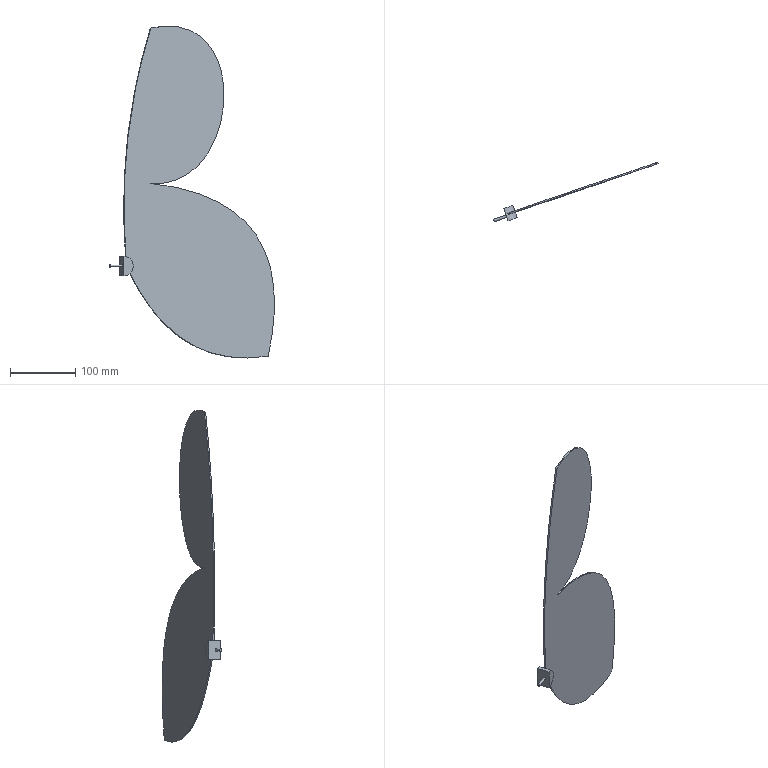Component | SolidWorks | Wing-1 | 1 solid | 13 faces | box 252.98 x 91.52 x 509.37 mm | volume 165544 mm3 | plane 6 | spline 4 | cylinder 3 | commonest cylinder face diameters 4 x2 30 x1
build123d program:
from build123d import *

# Parameters (mm, degrees)
BOSS_EXTRUDE1_DEPTH = 20
SKETCH25_R          = 2
BOSS_EXTRUDE3_DEPTH = 20
THICKEN1_T1         = 1
THICKEN1_T2         = 1


with BuildPart() as part:
    # Sketch1 → Boss-Extrude1 (new body)
    with BuildSketch(Plane.XY):
        with BuildLine():
            Line((-18.452, 20.731), (11.548, 20.731))
            ThreePointArc((11.548, 20.731), (-3.452, 5.731), (-18.452, 20.731))
        make_face()
    extrude(amount=BOSS_EXTRUDE1_DEPTH)

    # Sketch25 → Boss-Extrude3 (add)
    with BuildSketch(Plane(origin=(0, 20.731, 0), x_dir=(1, 0, 0), z_dir=(0, 1, 0))):
        with Locations(Location((-3.452, -7.5, 0), (0, 0, 90))):
            Circle(SKETCH25_R)
    extrude(amount=BOSS_EXTRUDE3_DEPTH)

    # Sketch26 → Surface-Plane2: a flat surface bounded by the sketch
    with BuildSketch(Plane.XY.offset(10), mode=Mode.PRIVATE) as surface_plane2_1_region:
        with BuildLine():
            add(Edge.make_bspline(
                [(-3.452, 13.231), (-191.154, 31.452), (-368.628, -25.683)],
                knots=[0, 0, 0, 1, 1, 1], degree=2))
            add(Edge.make_bspline(
                [(-368.628, -25.683), (-405.477, -194.567), (-118.532, -173.653), (-130.389, -25.683)],
                knots=[0, 0, 0, 0, 1, 1, 1, 1], degree=3))
            add(Edge.make_bspline(
                [(134.886, -216.099), (-105.129, -271.91), (-130.389, -25.683)],
                knots=[0, 0, 0, 1, 1, 1], degree=2))
            add(Edge.make_bspline(
                [(-3.452, 13.231), (156.545, -62.034), (134.886, -216.099)],
                knots=[0, 0, 0, 1, 1, 1], degree=2))
        make_face()
    surface_plane2_1 = surface_plane2_1_region.sketch.faces()[0]
    add(Solid.thicken(surface_plane2_1, THICKEN1_T1))
    add(Solid.thicken(surface_plane2_1, -THICKEN1_T2))


solid = part.part

# Placed as in the assembly
solid = solid.moved(Location((86.945, 39.336, 123.394), (-90, -18.851, 90)))
STEP:
#1=CARTESIAN_POINT('',(1.785,1.384,4.994));
#2=VERTEX_POINT('',#1);
#3=CARTESIAN_POINT('',(1.835,1.235,4.994));
#4=VERTEX_POINT('',#3);
#5=CARTESIAN_POINT('',(1.81,1.31,4.994));
#6=DIRECTION('',(-0.9464,-0.3231,0.));
#7=DIRECTION('',(-0.3231,0.9464,0.));
#8=AXIS2_PLACEMENT_3D('',#5,#6,#7);
#9=CIRCLE('',#8,0.07874);
#10=EDGE_CURVE('',#2,#4,#9,.T.);
#11=ORIENTED_EDGE('',*,*,#10,.F.);
#12=CARTESIAN_POINT('',(2.53,1.639,4.994));
#13=VERTEX_POINT('',#12);
#14=CARTESIAN_POINT('',(1.785,1.384,4.994));
#15=DIRECTION('',(0.9464,0.3231,-0.));
#16=VECTOR('',#15,39.37);
#17=LINE('',#14,#16);
#18=EDGE_CURVE('',#2,#13,#17,.T.);
#19=ORIENTED_EDGE('',*,*,#18,.T.);
#20=CARTESIAN_POINT('',(2.581,1.49,4.994));
#21=VERTEX_POINT('',#20);
#22=CARTESIAN_POINT('',(2.555,1.564,4.994));
#23=DIRECTION('',(-0.9464,-0.3231,0.));
#24=DIRECTION('',(0.3231,-0.9464,0.));
#25=AXIS2_PLACEMENT_3D('',#22,#23,#24);
#26=CIRCLE('',#25,0.07874);
#27=EDGE_CURVE('',#13,#21,#26,.T.);
#28=ORIENTED_EDGE('',*,*,#27,.T.);
#29=CARTESIAN_POINT('',(1.835,1.235,4.994));
#30=DIRECTION('',(0.9464,0.3231,-0.));
#31=VECTOR('',#30,39.37);
#32=LINE('',#29,#31);
#33=EDGE_CURVE('',#4,#21,#32,.T.);
#34=ORIENTED_EDGE('',*,*,#33,.F.);
#35=EDGE_LOOP('',(#11,#19,#28,#34));
#36=FACE_OUTER_BOUND('',#35,.T.);
#37=CARTESIAN_POINT('',(1.81,1.31,4.994));
#38=DIRECTION('',(0.9464,0.3231,-0.));
#39=DIRECTION('',(0.3231,-0.9464,0.));
#40=AXIS2_PLACEMENT_3D('',#37,#38,#39);
#41=CYLINDRICAL_SURFACE('',#40,0.07874);
#42=ADVANCED_FACE('',(#36),#41,.T.);
#43=CARTESIAN_POINT('',(2.77,1.7,5.53));
#44=VERTEX_POINT('',#43);
#45=CARTESIAN_POINT('',(2.745,1.775,5.53));
#46=VERTEX_POINT('',#45);
#47=CARTESIAN_POINT('',(2.757,1.737,5.53));
#48=DIRECTION('',(-0.3231,0.9464,0.));
#49=VECTOR('',#48,39.37);
#50=LINE('',#47,#49);
#51=EDGE_CURVE('',#44,#46,#50,.T.);
#52=ORIENTED_EDGE('',*,*,#51,.T.);
#53=CARTESIAN_POINT('',(2.955,1.846,4.635));
#54=VERTEX_POINT('',#53);
#55=CARTESIAN_POINT('',(2.511,1.695,4.994));
#56=DIRECTION('',(-0.3231,0.9464,0.));
#57=DIRECTION('',(0.,0.,-1.));
#58=AXIS2_PLACEMENT_3D('',#55,#56,#57);
#59=CIRCLE('',#58,0.5906);
#60=EDGE_CURVE('',#46,#54,#59,.T.);
#61=ORIENTED_EDGE('',*,*,#60,.T.);
#62=CARTESIAN_POINT('',(2.98,1.772,4.635));
#63=VERTEX_POINT('',#62);
#64=CARTESIAN_POINT('',(2.968,1.809,4.635));
#65=DIRECTION('',(0.3231,-0.9464,-0.));
#66=VECTOR('',#65,39.37);
#67=LINE('',#64,#66);
#68=EDGE_CURVE('',#54,#63,#67,.T.);
#69=ORIENTED_EDGE('',*,*,#68,.T.);
#70=CARTESIAN_POINT('',(2.536,1.62,4.994));
#71=DIRECTION('',(-0.3231,0.9464,0.));
#72=DIRECTION('',(0.,0.,-1.));
#73=AXIS2_PLACEMENT_3D('',#70,#71,#72);
#74=CIRCLE('',#73,0.5906);
#75=EDGE_CURVE('',#44,#63,#74,.T.);
#76=ORIENTED_EDGE('',*,*,#75,.F.);
#77=EDGE_LOOP('',(#52,#61,#69,#76));
#78=FACE_BOUND('',#77,.T.);
#79=CARTESIAN_POINT('',(2.651,1.285,5.584));
#80=VERTEX_POINT('',#79);
#81=CARTESIAN_POINT('',(2.651,1.285,4.403));
#82=VERTEX_POINT('',#81);
#83=CARTESIAN_POINT('',(2.651,1.285,4.994));
#84=DIRECTION('',(-0.3231,0.9464,0.));
#85=DIRECTION('',(0.,0.,-1.));
#86=AXIS2_PLACEMENT_3D('',#83,#84,#85);
#87=CIRCLE('',#86,0.5906);
#88=EDGE_CURVE('',#80,#82,#87,.T.);
#89=ORIENTED_EDGE('',*,*,#88,.T.);
#90=CARTESIAN_POINT('',(2.396,2.03,4.403));
#91=VERTEX_POINT('',#90);
#92=CARTESIAN_POINT('',(2.396,2.03,4.403));
#93=DIRECTION('',(0.3231,-0.9464,-0.));
#94=VECTOR('',#93,39.37);
#95=LINE('',#92,#94);
#96=EDGE_CURVE('',#91,#82,#95,.T.);
#97=ORIENTED_EDGE('',*,*,#96,.F.);
#98=CARTESIAN_POINT('',(2.396,2.03,5.584));
#99=VERTEX_POINT('',#98);
#100=CARTESIAN_POINT('',(2.396,2.03,4.994));
#101=DIRECTION('',(-0.3231,0.9464,0.));
#102=DIRECTION('',(0.,0.,-1.));
#103=AXIS2_PLACEMENT_3D('',#100,#101,#102);
#104=CIRCLE('',#103,0.5906);
#105=EDGE_CURVE('',#99,#91,#104,.T.);
#106=ORIENTED_EDGE('',*,*,#105,.F.);
#107=CARTESIAN_POINT('',(2.396,2.03,5.584));
#108=DIRECTION('',(0.3231,-0.9464,-0.));
#109=VECTOR('',#108,39.37);
#110=LINE('',#107,#109);
#111=EDGE_CURVE('',#99,#80,#110,.T.);
#112=ORIENTED_EDGE('',*,*,#111,.T.);
#113=EDGE_LOOP('',(#89,#97,#106,#112));
#114=FACE_OUTER_BOUND('',#113,.T.);
#115=CARTESIAN_POINT('',(2.396,2.03,4.994));
#116=DIRECTION('',(0.3231,-0.9464,-0.));
#117=DIRECTION('',(0.,0.,1.));
#118=AXIS2_PLACEMENT_3D('',#115,#116,#117);
#119=CYLINDRICAL_SURFACE('',#118,0.5906);
#120=ADVANCED_FACE('',(#78,#114),#119,.T.);
#121=CARTESIAN_POINT('',(2.555,1.564,4.994));
#122=DIRECTION('',(-0.9464,-0.3231,0.));
#123=DIRECTION('',(0.3231,-0.9464,0.));
#124=AXIS2_PLACEMENT_3D('',#121,#122,#123);
#125=CIRCLE('',#124,0.07874);
#126=EDGE_CURVE('',#21,#13,#125,.T.);
#127=ORIENTED_EDGE('',*,*,#126,.F.);
#128=ORIENTED_EDGE('',*,*,#27,.F.);
#129=EDGE_LOOP('',(#127,#128));
#130=FACE_BOUND('',#129,.T.);
#131=CARTESIAN_POINT('',(2.651,1.285,5.584));
#132=DIRECTION('',(0.,-0.,1.));
#133=VECTOR('',#132,39.37);
#134=LINE('',#131,#133);
#135=EDGE_CURVE('',#82,#80,#134,.T.);
#136=ORIENTED_EDGE('',*,*,#135,.T.);
#137=ORIENTED_EDGE('',*,*,#111,.F.);
#138=CARTESIAN_POINT('',(2.396,2.03,5.584));
#139=DIRECTION('',(0.,-0.,1.));
#140=VECTOR('',#139,39.37);
#141=LINE('',#138,#140);
#142=EDGE_CURVE('',#91,#99,#141,.T.);
#143=ORIENTED_EDGE('',*,*,#142,.F.);
#144=ORIENTED_EDGE('',*,*,#96,.T.);
#145=EDGE_LOOP('',(#136,#137,#143,#144));
#146=FACE_OUTER_BOUND('',#145,.T.);
#147=CARTESIAN_POINT('',(2.396,2.03,5.584));
#148=DIRECTION('',(0.9464,0.3231,-0.));
#149=DIRECTION('',(0.3231,-0.9464,-0.));
#150=AXIS2_PLACEMENT_3D('',#147,#148,#149);
#151=PLANE('',#150);
#152=ADVANCED_FACE('',(#130,#146),#151,.F.);
#153=ORIENTED_EDGE('',*,*,#105,.T.);
#154=ORIENTED_EDGE('',*,*,#142,.T.);
#155=EDGE_LOOP('',(#153,#154));
#156=FACE_OUTER_BOUND('',#155,.T.);
#157=CARTESIAN_POINT('',(2.396,2.03,4.994));
#158=DIRECTION('',(-0.3231,0.9464,0.));
#159=DIRECTION('',(-0.,0.,-1.));
#160=AXIS2_PLACEMENT_3D('',#157,#158,#159);
#161=PLANE('',#160);
#162=ADVANCED_FACE('',(#156),#161,.T.);
#163=ORIENTED_EDGE('',*,*,#88,.F.);
#164=ORIENTED_EDGE('',*,*,#135,.F.);
#165=EDGE_LOOP('',(#163,#164));
#166=FACE_OUTER_BOUND('',#165,.T.);
#167=CARTESIAN_POINT('',(2.651,1.285,4.994));
#168=DIRECTION('',(-0.3231,0.9464,0.));
#169=DIRECTION('',(-0.,0.,-1.));
#170=AXIS2_PLACEMENT_3D('',#167,#168,#169);
#171=PLANE('',#170);
#172=ADVANCED_FACE('',(#166),#171,.F.);
#173=ORIENTED_EDGE('',*,*,#18,.F.);
#174=CARTESIAN_POINT('',(1.81,1.31,4.994));
#175=DIRECTION('',(-0.9464,-0.3231,0.));
#176=DIRECTION('',(-0.3231,0.9464,0.));
#177=AXIS2_PLACEMENT_3D('',#174,#175,#176);
#178=CIRCLE('',#177,0.07874);
#179=EDGE_CURVE('',#4,#2,#178,.T.);
#180=ORIENTED_EDGE('',*,*,#179,.F.);
#181=ORIENTED_EDGE('',*,*,#33,.T.);
#182=ORIENTED_EDGE('',*,*,#126,.T.);
#183=EDGE_LOOP('',(#173,#180,#181,#182));
#184=FACE_OUTER_BOUND('',#183,.T.);
#185=CARTESIAN_POINT('',(1.81,1.31,4.994));
#186=DIRECTION('',(0.9464,0.3231,-0.));
#187=DIRECTION('',(0.3231,-0.9464,0.));
#188=AXIS2_PLACEMENT_3D('',#185,#186,#187);
#189=CYLINDRICAL_SURFACE('',#188,0.07874);
#190=ADVANCED_FACE('',(#184),#189,.T.);
#191=ORIENTED_EDGE('',*,*,#179,.T.);
#192=ORIENTED_EDGE('',*,*,#10,.T.);
#193=EDGE_LOOP('',(#191,#192));
#194=FACE_OUTER_BOUND('',#193,.T.);
#195=CARTESIAN_POINT('',(1.81,1.31,4.994));
#196=DIRECTION('',(-0.9464,-0.3231,0.));
#197=DIRECTION('',(-0.3231,0.9464,0.));
#198=AXIS2_PLACEMENT_3D('',#195,#196,#197);
#199=PLANE('',#198);
#200=ADVANCED_FACE('',(#194),#199,.T.);
#201=ORIENTED_EDGE('',*,*,#68,.F.);
#202=CARTESIAN_POINT('',(11.335,4.707,-0.4525));
#203=VERTEX_POINT('',#202);
#204=CARTESIAN_POINT('',(11.335,4.707,-0.4525));
#205=CARTESIAN_POINT('',(5.76,2.804,-1.281));
#206=CARTESIAN_POINT('',(2.955,1.846,4.635));
#207=B_SPLINE_CURVE_WITH_KNOTS('',2,(#204,#205,#206),.UNSPECIFIED.,.F.,.F.,(3,3),(0.,0.9711),.UNSPECIFIED.);
#208=EDGE_CURVE('',#203,#54,#207,.T.);
#209=ORIENTED_EDGE('',*,*,#208,.F.);
#210=CARTESIAN_POINT('',(11.36,4.633,-0.4525));
#211=VERTEX_POINT('',#210);
#212=CARTESIAN_POINT('',(11.347,4.67,-0.4525));
#213=DIRECTION('',(-0.3231,0.9464,0.));
#214=VECTOR('',#213,39.37);
#215=LINE('',#212,#214);
#216=EDGE_CURVE('',#211,#203,#215,.T.);
#217=ORIENTED_EDGE('',*,*,#216,.F.);
#218=CARTESIAN_POINT('',(11.36,4.633,-0.4525));
#219=CARTESIAN_POINT('',(5.786,2.73,-1.281));
#220=CARTESIAN_POINT('',(2.98,1.772,4.635));
#221=B_SPLINE_CURVE_WITH_KNOTS('',2,(#218,#219,#220),.UNSPECIFIED.,.F.,.F.,(3,3),(0.,0.9711),.UNSPECIFIED.);
#222=EDGE_CURVE('',#211,#63,#221,.T.);
#223=ORIENTED_EDGE('',*,*,#222,.T.);
#224=EDGE_LOOP('',(#201,#209,#217,#223));
#225=FACE_OUTER_BOUND('',#224,.T.);
#226=CARTESIAN_POINT('',(11.36,4.633,-0.4525));
#227=CARTESIAN_POINT('',(11.335,4.707,-0.4525));
#228=CARTESIAN_POINT('',(5.786,2.73,-1.281));
#229=CARTESIAN_POINT('',(5.76,2.804,-1.281));
#230=CARTESIAN_POINT('',(2.98,1.772,4.635));
#231=CARTESIAN_POINT('',(2.955,1.846,4.635));
#232=B_SPLINE_SURFACE_WITH_KNOTS('',2,1,((#226,#227),(#228,#229),(#230,#231)),.UNSPECIFIED.,.F.,.F.,.F.,(3,3),(2,2),(0.,0.9711),(0.,1.),.UNSPECIFIED.);
#233=ADVANCED_FACE('',(#225),#232,.T.);
#234=ORIENTED_EDGE('',*,*,#51,.F.);
#235=CARTESIAN_POINT('',(4.265,2.211,19.371));
#236=VERTEX_POINT('',#235);
#237=CARTESIAN_POINT('',(2.77,1.7,5.53));
#238=CARTESIAN_POINT('',(2.214,1.51,12.638));
#239=CARTESIAN_POINT('',(4.265,2.211,19.371));
#240=B_SPLINE_CURVE_WITH_KNOTS('',2,(#237,#238,#239),.UNSPECIFIED.,.F.,.F.,(3,3),(0.03633,1.),.UNSPECIFIED.);
#241=EDGE_CURVE('',#44,#236,#240,.T.);
#242=ORIENTED_EDGE('',*,*,#241,.T.);
#243=CARTESIAN_POINT('',(4.24,2.285,19.371));
#244=VERTEX_POINT('',#243);
#245=CARTESIAN_POINT('',(4.253,2.248,19.371));
#246=DIRECTION('',(-0.3231,0.9464,0.));
#247=VECTOR('',#246,39.37);
#248=LINE('',#245,#247);
#249=EDGE_CURVE('',#236,#244,#248,.T.);
#250=ORIENTED_EDGE('',*,*,#249,.T.);
#251=CARTESIAN_POINT('',(2.745,1.775,5.53));
#252=CARTESIAN_POINT('',(2.189,1.585,12.638));
#253=CARTESIAN_POINT('',(4.24,2.285,19.371));
#254=B_SPLINE_CURVE_WITH_KNOTS('',2,(#251,#252,#253),.UNSPECIFIED.,.F.,.F.,(3,3),(0.03633,1.),.UNSPECIFIED.);
#255=EDGE_CURVE('',#46,#244,#254,.T.);
#256=ORIENTED_EDGE('',*,*,#255,.F.);
#257=EDGE_LOOP('',(#234,#242,#250,#256));
#258=FACE_OUTER_BOUND('',#257,.T.);
#259=CARTESIAN_POINT('',(2.77,1.7,5.53));
#260=CARTESIAN_POINT('',(2.745,1.775,5.53));
#261=CARTESIAN_POINT('',(2.214,1.51,12.638));
#262=CARTESIAN_POINT('',(2.189,1.585,12.638));
#263=CARTESIAN_POINT('',(4.265,2.211,19.371));
#264=CARTESIAN_POINT('',(4.24,2.285,19.371));
#265=B_SPLINE_SURFACE_WITH_KNOTS('',2,1,((#259,#260),(#261,#262),(#263,#264)),.UNSPECIFIED.,.F.,.F.,.F.,(3,3),(2,2),(0.03633,1.),(0.,1.),.UNSPECIFIED.);
#266=ADVANCED_FACE('',(#258),#265,.T.);
#267=ORIENTED_EDGE('',*,*,#249,.F.);
#268=CARTESIAN_POINT('',(4.265,2.211,9.991));
#269=VERTEX_POINT('',#268);
#270=CARTESIAN_POINT('',(4.265,2.211,19.371));
#271=CARTESIAN_POINT('',(10.558,4.359,20.822));
#272=CARTESIAN_POINT('',(9.779,4.093,9.525));
#273=CARTESIAN_POINT('',(4.265,2.211,9.991));
#274=B_SPLINE_CURVE_WITH_KNOTS('',3,(#270,#271,#272,#273),.UNSPECIFIED.,.F.,.F.,(4,4),(0.,1.),.UNSPECIFIED.);
#275=EDGE_CURVE('',#236,#269,#274,.T.);
#276=ORIENTED_EDGE('',*,*,#275,.T.);
#277=CARTESIAN_POINT('',(4.24,2.285,9.991));
#278=VERTEX_POINT('',#277);
#279=CARTESIAN_POINT('',(4.253,2.248,9.991));
#280=DIRECTION('',(-0.3231,0.9464,0.));
#281=VECTOR('',#280,39.37);
#282=LINE('',#279,#281);
#283=EDGE_CURVE('',#269,#278,#282,.T.);
#284=ORIENTED_EDGE('',*,*,#283,.T.);
#285=CARTESIAN_POINT('',(4.24,2.285,19.371));
#286=CARTESIAN_POINT('',(10.532,4.434,20.822));
#287=CARTESIAN_POINT('',(9.753,4.167,9.525));
#288=CARTESIAN_POINT('',(4.24,2.285,9.991));
#289=B_SPLINE_CURVE_WITH_KNOTS('',3,(#285,#286,#287,#288),.UNSPECIFIED.,.F.,.F.,(4,4),(0.,1.),.UNSPECIFIED.);
#290=EDGE_CURVE('',#244,#278,#289,.T.);
#291=ORIENTED_EDGE('',*,*,#290,.F.);
#292=EDGE_LOOP('',(#267,#276,#284,#291));
#293=FACE_OUTER_BOUND('',#292,.T.);
#294=CARTESIAN_POINT('',(4.265,2.211,19.371));
#295=CARTESIAN_POINT('',(4.24,2.285,19.371));
#296=CARTESIAN_POINT('',(10.558,4.359,20.822));
#297=CARTESIAN_POINT('',(10.532,4.434,20.822));
#298=CARTESIAN_POINT('',(9.779,4.093,9.525));
#299=CARTESIAN_POINT('',(9.753,4.167,9.525));
#300=CARTESIAN_POINT('',(4.265,2.211,9.991));
#301=CARTESIAN_POINT('',(4.24,2.285,9.991));
#302=B_SPLINE_SURFACE_WITH_KNOTS('',3,1,((#294,#295),(#296,#297),(#298,#299),(#300,#301)),.UNSPECIFIED.,.F.,.F.,.F.,(4,4),(2,2),(0.,1.),(0.,1.),.UNSPECIFIED.);
#303=ADVANCED_FACE('',(#293),#302,.T.);
#304=ORIENTED_EDGE('',*,*,#283,.F.);
#305=CARTESIAN_POINT('',(4.265,2.211,9.991));
#306=CARTESIAN_POINT('',(13.439,5.343,8.997));
#307=CARTESIAN_POINT('',(11.36,4.633,-0.4525));
#308=B_SPLINE_CURVE_WITH_KNOTS('',2,(#305,#306,#307),.UNSPECIFIED.,.F.,.F.,(3,3),(0.,1.),.UNSPECIFIED.);
#309=EDGE_CURVE('',#269,#211,#308,.T.);
#310=ORIENTED_EDGE('',*,*,#309,.T.);
#311=ORIENTED_EDGE('',*,*,#216,.T.);
#312=CARTESIAN_POINT('',(4.24,2.285,9.991));
#313=CARTESIAN_POINT('',(13.414,5.417,8.997));
#314=CARTESIAN_POINT('',(11.335,4.707,-0.4525));
#315=B_SPLINE_CURVE_WITH_KNOTS('',2,(#312,#313,#314),.UNSPECIFIED.,.F.,.F.,(3,3),(0.,1.),.UNSPECIFIED.);
#316=EDGE_CURVE('',#278,#203,#315,.T.);
#317=ORIENTED_EDGE('',*,*,#316,.F.);
#318=EDGE_LOOP('',(#304,#310,#311,#317));
#319=FACE_OUTER_BOUND('',#318,.T.);
#320=CARTESIAN_POINT('',(4.265,2.211,9.991));
#321=CARTESIAN_POINT('',(4.24,2.285,9.991));
#322=CARTESIAN_POINT('',(13.439,5.343,8.997));
#323=CARTESIAN_POINT('',(13.414,5.417,8.997));
#324=CARTESIAN_POINT('',(11.36,4.633,-0.4525));
#325=CARTESIAN_POINT('',(11.335,4.707,-0.4525));
#326=B_SPLINE_SURFACE_WITH_KNOTS('',2,1,((#320,#321),(#322,#323),(#324,#325)),.UNSPECIFIED.,.F.,.F.,.F.,(3,3),(2,2),(0.,1.),(0.,1.),.UNSPECIFIED.);
#327=ADVANCED_FACE('',(#319),#326,.T.);
#328=ORIENTED_EDGE('',*,*,#60,.F.);
#329=ORIENTED_EDGE('',*,*,#255,.T.);
#330=ORIENTED_EDGE('',*,*,#290,.T.);
#331=ORIENTED_EDGE('',*,*,#316,.T.);
#332=ORIENTED_EDGE('',*,*,#208,.T.);
#333=EDGE_LOOP('',(#328,#329,#330,#331,#332));
#334=FACE_OUTER_BOUND('',#333,.T.);
#335=CARTESIAN_POINT('',(6.328,2.998,0.4828));
#336=DIRECTION('',(-0.3231,0.9464,0.));
#337=DIRECTION('',(-0.,0.,-1.));
#338=AXIS2_PLACEMENT_3D('',#335,#336,#337);
#339=PLANE('',#338);
#340=ADVANCED_FACE('',(#334),#339,.T.);
#341=ORIENTED_EDGE('',*,*,#241,.F.);
#342=ORIENTED_EDGE('',*,*,#75,.T.);
#343=ORIENTED_EDGE('',*,*,#222,.F.);
#344=ORIENTED_EDGE('',*,*,#309,.F.);
#345=ORIENTED_EDGE('',*,*,#275,.F.);
#346=EDGE_LOOP('',(#341,#342,#343,#344,#345));
#347=FACE_OUTER_BOUND('',#346,.T.);
#348=CARTESIAN_POINT('',(6.354,2.924,0.4828));
#349=DIRECTION('',(-0.3231,0.9464,0.));
#350=DIRECTION('',(-0.,0.,-1.));
#351=AXIS2_PLACEMENT_3D('',#348,#349,#350);
#352=PLANE('',#351);
#353=ADVANCED_FACE('',(#347),#352,.F.);
#354=CLOSED_SHELL('',(#42,#120,#152,#162,#172,#190,#200,#233,#266,#303,#327,#340,#353));
#355=MANIFOLD_SOLID_BREP('',#354);
#356=CARTESIAN_POINT('',(0.,0.,0.));
#357=DIRECTION('',(0.,0.,1.));
#358=DIRECTION('',(1.,0.,0.));
#359=AXIS2_PLACEMENT_3D('',#356,#357,#358);
#360=(LENGTH_UNIT()NAMED_UNIT(*)SI_UNIT($,.METRE.));
#361=LENGTH_MEASURE_WITH_UNIT(LENGTH_MEASURE(0.0254),#360);
#362=DIMENSIONAL_EXPONENTS(1.,0.,0.,0.,0.,0.,0.);
#363=(CONVERSION_BASED_UNIT('',#361)LENGTH_UNIT()NAMED_UNIT(#362));
#364=UNCERTAINTY_MEASURE_WITH_UNIT(LENGTH_MEASURE(0.00001),#363,'','');
#365=(NAMED_UNIT(*)PLANE_ANGLE_UNIT()SI_UNIT($,.RADIAN.));
#366=(NAMED_UNIT(*)SI_UNIT($,.STERADIAN.)SOLID_ANGLE_UNIT());
#367=(GEOMETRIC_REPRESENTATION_CONTEXT(3)GLOBAL_UNCERTAINTY_ASSIGNED_CONTEXT((#364))GLOBAL_UNIT_ASSIGNED_CONTEXT((#363,#365,#366))REPRESENTATION_CONTEXT('',''));
#368=ADVANCED_BREP_SHAPE_REPRESENTATION('',(#355,#359),#367);
#369=COLOUR_RGB('',0.7922,0.8196,0.9333);
#370=FILL_AREA_STYLE_COLOUR('',#369);
#371=FILL_AREA_STYLE('',(#370));
#372=SURFACE_STYLE_FILL_AREA(#371);
#373=SURFACE_SIDE_STYLE('',(#372));
#374=SURFACE_STYLE_USAGE(.BOTH.,#373);
#375=PRESENTATION_STYLE_ASSIGNMENT((#374));
#376=STYLED_ITEM('',(#375),#355);
#377=PRESENTATION_LAYER_ASSIGNMENT('','',(#376));
#378=(LENGTH_UNIT()NAMED_UNIT(*)SI_UNIT($,.METRE.));
#379=LENGTH_MEASURE_WITH_UNIT(LENGTH_MEASURE(0.0254),#378);
#380=DIMENSIONAL_EXPONENTS(1.,0.,0.,0.,0.,0.,0.);
#381=(CONVERSION_BASED_UNIT('',#379)LENGTH_UNIT()NAMED_UNIT(#380));
#382=UNCERTAINTY_MEASURE_WITH_UNIT(LENGTH_MEASURE(0.00001),#381,'','');
#383=(NAMED_UNIT(*)PLANE_ANGLE_UNIT()SI_UNIT($,.RADIAN.));
#384=(NAMED_UNIT(*)SI_UNIT($,.STERADIAN.)SOLID_ANGLE_UNIT());
#385=(GEOMETRIC_REPRESENTATION_CONTEXT(3)GLOBAL_UNCERTAINTY_ASSIGNED_CONTEXT((#382))GLOBAL_UNIT_ASSIGNED_CONTEXT((#381,#383,#384))REPRESENTATION_CONTEXT('',''));
#386=MECHANICAL_DESIGN_GEOMETRIC_PRESENTATION_REPRESENTATION('',(#376),#385);